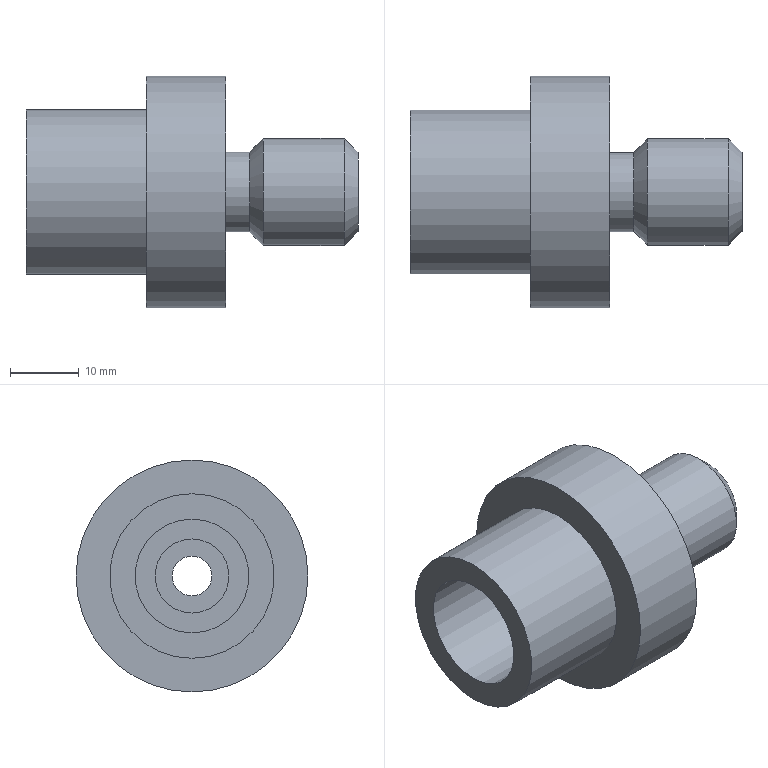Component | NX | VALVE_PORT | 1 solid | 15 faces | box 48.4 x 33.8 x 33.8 mm | volume 16682 mm3 | cylinder 7 | plane 6 | cone 2 | commonest cylinder face diameters 5.8 x1 10.8 x1 16.6 x1 24 x1 33.8 x1 11.6 x1 15.6 x1
STEP:
#1=CARTESIAN_POINT('',(0.,0.,0.));
#2=DIRECTION('',(0.,0.,1.));
#3=DIRECTION('',(1.,0.,0.));
#4=AXIS2_PLACEMENT_3D('',#1,#2,#3);
#5=CARTESIAN_POINT('',(119.195,-20.891,-5.8));
#6=VERTEX_POINT('',#5);
#7=CARTESIAN_POINT('',(119.195,-20.891,0.));
#8=DIRECTION('',(1.,0.,0.));
#9=DIRECTION('',(0.,0.,-1.));
#10=AXIS2_PLACEMENT_3D('',#7,#8,#9);
#11=CIRCLE('',#10,5.8);
#12=CARTESIAN_POINT('',(119.195,-28.691,0.));
#13=DIRECTION('',(-1.,0.,0.));
#14=DIRECTION('',(0.,0.,-1.));
#15=AXIS2_PLACEMENT_3D('',#12,#13,#14);
#16=PLANE('',#15);
#17=CARTESIAN_POINT('',(5.8,-7.8));
#18=CARTESIAN_POINT('',(5.8,-17.846));
#19=CARTESIAN_POINT('',(-2.9,-12.823));
#20=CARTESIAN_POINT('',(-11.6,-7.8));
#21=CARTESIAN_POINT('',(-2.9,-2.777));
#22=CARTESIAN_POINT('',(5.8,2.246));
#23=CARTESIAN_POINT('',(5.8,-7.8));
#24=(BOUNDED_CURVE()B_SPLINE_CURVE(2,(#17,#18,#19,#20,#21,#22,#23),.UNSPECIFIED.,.T.,.F.)B_SPLINE_CURVE_WITH_KNOTS((1,2,2,2,2,1),(-2.094,0.,2.094,4.189,6.283,8.378),.UNSPECIFIED.)CURVE()GEOMETRIC_REPRESENTATION_ITEM()RATIONAL_B_SPLINE_CURVE((1.,0.5,1.,0.5,1.,0.5,1.))REPRESENTATION_ITEM(''));
#25=(GEOMETRIC_REPRESENTATION_CONTEXT(2)PARAMETRIC_REPRESENTATION_CONTEXT()REPRESENTATION_CONTEXT('',''));
#26=DEFINITIONAL_REPRESENTATION('',(#24),#25);
#27=PCURVE('',#16,#26);
#28=CARTESIAN_POINT('',(119.195,-20.891,0.));
#29=DIRECTION('',(-1.,0.,0.));
#30=DIRECTION('',(0.,0.,-1.));
#31=AXIS2_PLACEMENT_3D('',#28,#29,#30);
#32=CONICAL_SURFACE('',#31,5.8,0.7854);
#33=CARTESIAN_POINT('',(6.283,0.));
#34=DIRECTION('',(-1.,0.));
#35=VECTOR('',#34,1.);
#36=LINE('',#33,#35);
#37=(GEOMETRIC_REPRESENTATION_CONTEXT(2)PARAMETRIC_REPRESENTATION_CONTEXT()REPRESENTATION_CONTEXT('',''));
#38=DEFINITIONAL_REPRESENTATION('',(#36),#37);
#39=PCURVE('',#32,#38);
#40=SURFACE_CURVE('',#11,(#27,#39),.PCURVE_S1.);
#41=EDGE_CURVE('',#6,#6,#40,.T.);
#42=ORIENTED_EDGE('',*,*,#41,.T.);
#43=EDGE_LOOP('',(#42));
#44=FACE_BOUND('',#43,.T.);
#45=CARTESIAN_POINT('',(119.195,-20.891,2.9));
#46=VERTEX_POINT('',#45);
#47=CARTESIAN_POINT('',(119.195,-20.891,0.));
#48=DIRECTION('',(1.,0.,0.));
#49=DIRECTION('',(0.,0.,1.));
#50=AXIS2_PLACEMENT_3D('',#47,#48,#49);
#51=CIRCLE('',#50,2.9);
#52=CARTESIAN_POINT('',(-2.9,-7.8));
#53=CARTESIAN_POINT('',(-2.9,-2.777));
#54=CARTESIAN_POINT('',(1.45,-5.289));
#55=CARTESIAN_POINT('',(5.8,-7.8));
#56=CARTESIAN_POINT('',(1.45,-10.311));
#57=CARTESIAN_POINT('',(-2.9,-12.823));
#58=CARTESIAN_POINT('',(-2.9,-7.8));
#59=(BOUNDED_CURVE()B_SPLINE_CURVE(2,(#52,#53,#54,#55,#56,#57,#58),.UNSPECIFIED.,.T.,.F.)B_SPLINE_CURVE_WITH_KNOTS((1,2,2,2,2,1),(-2.094,0.,2.094,4.189,6.283,8.378),.UNSPECIFIED.)CURVE()GEOMETRIC_REPRESENTATION_ITEM()RATIONAL_B_SPLINE_CURVE((1.,0.5,1.,0.5,1.,0.5,1.))REPRESENTATION_ITEM(''));
#60=(GEOMETRIC_REPRESENTATION_CONTEXT(2)PARAMETRIC_REPRESENTATION_CONTEXT()REPRESENTATION_CONTEXT('',''));
#61=DEFINITIONAL_REPRESENTATION('',(#59),#60);
#62=PCURVE('',#16,#61);
#63=CARTESIAN_POINT('',(70.795,-20.891,0.));
#64=DIRECTION('',(1.,0.,0.));
#65=DIRECTION('',(0.,0.,1.));
#66=AXIS2_PLACEMENT_3D('',#63,#64,#65);
#67=CYLINDRICAL_SURFACE('',#66,2.9);
#68=CARTESIAN_POINT('',(0.,48.4));
#69=DIRECTION('',(1.,0.));
#70=VECTOR('',#69,1.);
#71=LINE('',#68,#70);
#72=(GEOMETRIC_REPRESENTATION_CONTEXT(2)PARAMETRIC_REPRESENTATION_CONTEXT()REPRESENTATION_CONTEXT('',''));
#73=DEFINITIONAL_REPRESENTATION('',(#71),#72);
#74=PCURVE('',#67,#73);
#75=SURFACE_CURVE('',#51,(#62,#74),.PCURVE_S1.);
#76=EDGE_CURVE('',#46,#46,#75,.T.);
#77=ORIENTED_EDGE('',*,*,#76,.F.);
#78=EDGE_LOOP('',(#77));
#79=FACE_BOUND('',#78,.T.);
#80=ADVANCED_FACE('',(#44,#79),#16,.F.);
#81=CARTESIAN_POINT('',(88.295,-20.891,2.9));
#82=VERTEX_POINT('',#81);
#83=CARTESIAN_POINT('',(88.295,-20.891,0.));
#84=DIRECTION('',(1.,0.,0.));
#85=DIRECTION('',(0.,0.,1.));
#86=AXIS2_PLACEMENT_3D('',#83,#84,#85);
#87=CIRCLE('',#86,2.9);
#88=CARTESIAN_POINT('',(0.,17.5));
#89=DIRECTION('',(1.,0.));
#90=VECTOR('',#89,1.);
#91=LINE('',#88,#90);
#92=(GEOMETRIC_REPRESENTATION_CONTEXT(2)PARAMETRIC_REPRESENTATION_CONTEXT()REPRESENTATION_CONTEXT('',''));
#93=DEFINITIONAL_REPRESENTATION('',(#91),#92);
#94=PCURVE('',#67,#93);
#95=CARTESIAN_POINT('',(88.295,-23.791,0.));
#96=DIRECTION('',(1.,0.,0.));
#97=DIRECTION('',(0.,0.,1.));
#98=AXIS2_PLACEMENT_3D('',#95,#96,#97);
#99=PLANE('',#98);
#100=CARTESIAN_POINT('',(0.,-2.9));
#101=DIRECTION('',(1.,0.));
#102=AXIS2_PLACEMENT_2D('',#100,#101);
#103=CIRCLE('',#102,2.9);
#104=(GEOMETRIC_REPRESENTATION_CONTEXT(2)PARAMETRIC_REPRESENTATION_CONTEXT()REPRESENTATION_CONTEXT('',''));
#105=DEFINITIONAL_REPRESENTATION('',(#103),#104);
#106=PCURVE('',#99,#105);
#107=SURFACE_CURVE('',#87,(#94,#106),.PCURVE_S1.);
#108=EDGE_CURVE('',#82,#82,#107,.T.);
#109=ORIENTED_EDGE('',*,*,#108,.T.);
#110=CARTESIAN_POINT('',(88.295,-20.891,2.9));
#111=CARTESIAN_POINT('',(119.195,-20.891,2.9));
#112=B_SPLINE_CURVE_WITH_KNOTS('',1,(#110,#111),.UNSPECIFIED.,.F.,.F.,(2,2),(17.5,48.4),.PIECEWISE_BEZIER_KNOTS.);
#113=CARTESIAN_POINT('',(6.283,0.));
#114=DIRECTION('',(0.,1.));
#115=VECTOR('',#114,1.);
#116=LINE('',#113,#115);
#117=(GEOMETRIC_REPRESENTATION_CONTEXT(2)PARAMETRIC_REPRESENTATION_CONTEXT()REPRESENTATION_CONTEXT('',''));
#118=DEFINITIONAL_REPRESENTATION('',(#116),#117);
#119=PCURVE('',#67,#118);
#120=CARTESIAN_POINT('',(0.,0.));
#121=DIRECTION('',(0.,1.));
#122=VECTOR('',#121,1.);
#123=LINE('',#120,#122);
#124=(GEOMETRIC_REPRESENTATION_CONTEXT(2)PARAMETRIC_REPRESENTATION_CONTEXT()REPRESENTATION_CONTEXT('',''));
#125=DEFINITIONAL_REPRESENTATION('',(#123),#124);
#126=PCURVE('',#67,#125);
#127=SEAM_CURVE('',#112,(#119,#126),.PCURVE_S1.);
#128=EDGE_CURVE('',#82,#46,#127,.T.);
#129=ORIENTED_EDGE('',*,*,#128,.T.);
#130=ORIENTED_EDGE('',*,*,#76,.F.);
#131=ORIENTED_EDGE('',*,*,#128,.F.);
#132=EDGE_LOOP('',(#109,#129,#130,#131));
#133=FACE_BOUND('',#132,.F.);
#134=ADVANCED_FACE('',(#133),#67,.F.);
#135=CARTESIAN_POINT('',(88.295,-20.891,5.4));
#136=VERTEX_POINT('',#135);
#137=CARTESIAN_POINT('',(88.295,-20.891,0.));
#138=DIRECTION('',(1.,0.,0.));
#139=DIRECTION('',(0.,0.,1.));
#140=AXIS2_PLACEMENT_3D('',#137,#138,#139);
#141=CIRCLE('',#140,5.4);
#142=CARTESIAN_POINT('',(0.,-2.9));
#143=DIRECTION('',(1.,0.));
#144=AXIS2_PLACEMENT_2D('',#142,#143);
#145=CIRCLE('',#144,5.4);
#146=(GEOMETRIC_REPRESENTATION_CONTEXT(2)PARAMETRIC_REPRESENTATION_CONTEXT()REPRESENTATION_CONTEXT('',''));
#147=DEFINITIONAL_REPRESENTATION('',(#145),#146);
#148=PCURVE('',#99,#147);
#149=CARTESIAN_POINT('',(70.795,-20.891,0.));
#150=DIRECTION('',(1.,0.,0.));
#151=DIRECTION('',(0.,0.,1.));
#152=AXIS2_PLACEMENT_3D('',#149,#150,#151);
#153=CYLINDRICAL_SURFACE('',#152,5.4);
#154=CARTESIAN_POINT('',(0.,17.5));
#155=DIRECTION('',(1.,0.));
#156=VECTOR('',#155,1.);
#157=LINE('',#154,#156);
#158=(GEOMETRIC_REPRESENTATION_CONTEXT(2)PARAMETRIC_REPRESENTATION_CONTEXT()REPRESENTATION_CONTEXT('',''));
#159=DEFINITIONAL_REPRESENTATION('',(#157),#158);
#160=PCURVE('',#153,#159);
#161=SURFACE_CURVE('',#141,(#148,#160),.PCURVE_S1.);
#162=EDGE_CURVE('',#136,#136,#161,.T.);
#163=ORIENTED_EDGE('',*,*,#162,.F.);
#164=EDGE_LOOP('',(#163));
#165=FACE_BOUND('',#164,.T.);
#166=ORIENTED_EDGE('',*,*,#108,.T.);
#167=EDGE_LOOP('',(#166));
#168=FACE_BOUND('',#167,.T.);
#169=ADVANCED_FACE('',(#165,#168),#99,.F.);
#170=CARTESIAN_POINT('',(90.295,-20.891,5.4));
#171=VERTEX_POINT('',#170);
#172=CARTESIAN_POINT('',(90.295,-20.891,0.));
#173=DIRECTION('',(1.,0.,0.));
#174=DIRECTION('',(0.,0.,1.));
#175=AXIS2_PLACEMENT_3D('',#172,#173,#174);
#176=CIRCLE('',#175,5.4);
#177=CARTESIAN_POINT('',(0.,19.5));
#178=DIRECTION('',(1.,0.));
#179=VECTOR('',#178,1.);
#180=LINE('',#177,#179);
#181=(GEOMETRIC_REPRESENTATION_CONTEXT(2)PARAMETRIC_REPRESENTATION_CONTEXT()REPRESENTATION_CONTEXT('',''));
#182=DEFINITIONAL_REPRESENTATION('',(#180),#181);
#183=PCURVE('',#153,#182);
#184=CARTESIAN_POINT('',(90.295,-26.291,0.));
#185=DIRECTION('',(1.,0.,0.));
#186=DIRECTION('',(0.,0.,1.));
#187=AXIS2_PLACEMENT_3D('',#184,#185,#186);
#188=PLANE('',#187);
#189=CARTESIAN_POINT('',(0.,-5.4));
#190=DIRECTION('',(1.,0.));
#191=AXIS2_PLACEMENT_2D('',#189,#190);
#192=CIRCLE('',#191,5.4);
#193=(GEOMETRIC_REPRESENTATION_CONTEXT(2)PARAMETRIC_REPRESENTATION_CONTEXT()REPRESENTATION_CONTEXT('',''));
#194=DEFINITIONAL_REPRESENTATION('',(#192),#193);
#195=PCURVE('',#188,#194);
#196=SURFACE_CURVE('',#176,(#183,#195),.PCURVE_S1.);
#197=EDGE_CURVE('',#171,#171,#196,.T.);
#198=ORIENTED_EDGE('',*,*,#197,.F.);
#199=CARTESIAN_POINT('',(88.295,-20.891,5.4));
#200=CARTESIAN_POINT('',(90.295,-20.891,5.4));
#201=B_SPLINE_CURVE_WITH_KNOTS('',1,(#199,#200),.UNSPECIFIED.,.F.,.F.,(2,2),(17.5,19.5),.PIECEWISE_BEZIER_KNOTS.);
#202=CARTESIAN_POINT('',(0.,0.));
#203=DIRECTION('',(0.,1.));
#204=VECTOR('',#203,1.);
#205=LINE('',#202,#204);
#206=(GEOMETRIC_REPRESENTATION_CONTEXT(2)PARAMETRIC_REPRESENTATION_CONTEXT()REPRESENTATION_CONTEXT('',''));
#207=DEFINITIONAL_REPRESENTATION('',(#205),#206);
#208=PCURVE('',#153,#207);
#209=CARTESIAN_POINT('',(6.283,0.));
#210=DIRECTION('',(0.,1.));
#211=VECTOR('',#210,1.);
#212=LINE('',#209,#211);
#213=(GEOMETRIC_REPRESENTATION_CONTEXT(2)PARAMETRIC_REPRESENTATION_CONTEXT()REPRESENTATION_CONTEXT('',''));
#214=DEFINITIONAL_REPRESENTATION('',(#212),#213);
#215=PCURVE('',#153,#214);
#216=SEAM_CURVE('',#201,(#208,#215),.PCURVE_S1.);
#217=EDGE_CURVE('',#136,#171,#216,.T.);
#218=ORIENTED_EDGE('',*,*,#217,.F.);
#219=ORIENTED_EDGE('',*,*,#162,.T.);
#220=ORIENTED_EDGE('',*,*,#217,.T.);
#221=EDGE_LOOP('',(#198,#218,#219,#220));
#222=FACE_BOUND('',#221,.T.);
#223=ADVANCED_FACE('',(#222),#153,.T.);
#224=CARTESIAN_POINT('',(90.295,-20.891,8.3));
#225=VERTEX_POINT('',#224);
#226=CARTESIAN_POINT('',(90.295,-20.891,0.));
#227=DIRECTION('',(1.,0.,0.));
#228=DIRECTION('',(0.,0.,1.));
#229=AXIS2_PLACEMENT_3D('',#226,#227,#228);
#230=CIRCLE('',#229,8.3);
#231=CARTESIAN_POINT('',(0.,-5.4));
#232=DIRECTION('',(1.,0.));
#233=AXIS2_PLACEMENT_2D('',#231,#232);
#234=CIRCLE('',#233,8.3);
#235=(GEOMETRIC_REPRESENTATION_CONTEXT(2)PARAMETRIC_REPRESENTATION_CONTEXT()REPRESENTATION_CONTEXT('',''));
#236=DEFINITIONAL_REPRESENTATION('',(#234),#235);
#237=PCURVE('',#188,#236);
#238=CARTESIAN_POINT('',(70.795,-20.891,0.));
#239=DIRECTION('',(1.,0.,0.));
#240=DIRECTION('',(0.,0.,1.));
#241=AXIS2_PLACEMENT_3D('',#238,#239,#240);
#242=CYLINDRICAL_SURFACE('',#241,8.3);
#243=CARTESIAN_POINT('',(0.,19.5));
#244=DIRECTION('',(1.,0.));
#245=VECTOR('',#244,1.);
#246=LINE('',#243,#245);
#247=(GEOMETRIC_REPRESENTATION_CONTEXT(2)PARAMETRIC_REPRESENTATION_CONTEXT()REPRESENTATION_CONTEXT('',''));
#248=DEFINITIONAL_REPRESENTATION('',(#246),#247);
#249=PCURVE('',#242,#248);
#250=SURFACE_CURVE('',#230,(#237,#249),.PCURVE_S1.);
#251=EDGE_CURVE('',#225,#225,#250,.T.);
#252=ORIENTED_EDGE('',*,*,#251,.F.);
#253=EDGE_LOOP('',(#252));
#254=FACE_BOUND('',#253,.T.);
#255=ORIENTED_EDGE('',*,*,#197,.T.);
#256=EDGE_LOOP('',(#255));
#257=FACE_BOUND('',#256,.T.);
#258=ADVANCED_FACE('',(#254,#257),#188,.F.);
#259=CARTESIAN_POINT('',(70.795,-20.891,8.3));
#260=VERTEX_POINT('',#259);
#261=CARTESIAN_POINT('',(70.795,-20.891,0.));
#262=DIRECTION('',(1.,0.,0.));
#263=DIRECTION('',(0.,0.,1.));
#264=AXIS2_PLACEMENT_3D('',#261,#262,#263);
#265=CIRCLE('',#264,8.3);
#266=CARTESIAN_POINT('',(0.,0.));
#267=DIRECTION('',(1.,0.));
#268=VECTOR('',#267,1.);
#269=LINE('',#266,#268);
#270=(GEOMETRIC_REPRESENTATION_CONTEXT(2)PARAMETRIC_REPRESENTATION_CONTEXT()REPRESENTATION_CONTEXT('',''));
#271=DEFINITIONAL_REPRESENTATION('',(#269),#270);
#272=PCURVE('',#242,#271);
#273=CARTESIAN_POINT('',(70.795,-29.191,0.));
#274=DIRECTION('',(1.,0.,0.));
#275=DIRECTION('',(0.,0.,1.));
#276=AXIS2_PLACEMENT_3D('',#273,#274,#275);
#277=PLANE('',#276);
#278=CARTESIAN_POINT('',(0.,-8.3));
#279=DIRECTION('',(1.,0.));
#280=AXIS2_PLACEMENT_2D('',#278,#279);
#281=CIRCLE('',#280,8.3);
#282=(GEOMETRIC_REPRESENTATION_CONTEXT(2)PARAMETRIC_REPRESENTATION_CONTEXT()REPRESENTATION_CONTEXT('',''));
#283=DEFINITIONAL_REPRESENTATION('',(#281),#282);
#284=PCURVE('',#277,#283);
#285=SURFACE_CURVE('',#265,(#272,#284),.PCURVE_S1.);
#286=EDGE_CURVE('',#260,#260,#285,.T.);
#287=ORIENTED_EDGE('',*,*,#286,.T.);
#288=CARTESIAN_POINT('',(70.795,-20.891,8.3));
#289=CARTESIAN_POINT('',(90.295,-20.891,8.3));
#290=B_SPLINE_CURVE_WITH_KNOTS('',1,(#288,#289),.UNSPECIFIED.,.F.,.F.,(2,2),(0.,19.5),.PIECEWISE_BEZIER_KNOTS.);
#291=CARTESIAN_POINT('',(6.283,0.));
#292=DIRECTION('',(0.,1.));
#293=VECTOR('',#292,1.);
#294=LINE('',#291,#293);
#295=(GEOMETRIC_REPRESENTATION_CONTEXT(2)PARAMETRIC_REPRESENTATION_CONTEXT()REPRESENTATION_CONTEXT('',''));
#296=DEFINITIONAL_REPRESENTATION('',(#294),#295);
#297=PCURVE('',#242,#296);
#298=CARTESIAN_POINT('',(0.,0.));
#299=DIRECTION('',(0.,1.));
#300=VECTOR('',#299,1.);
#301=LINE('',#298,#300);
#302=(GEOMETRIC_REPRESENTATION_CONTEXT(2)PARAMETRIC_REPRESENTATION_CONTEXT()REPRESENTATION_CONTEXT('',''));
#303=DEFINITIONAL_REPRESENTATION('',(#301),#302);
#304=PCURVE('',#242,#303);
#305=SEAM_CURVE('',#290,(#297,#304),.PCURVE_S1.);
#306=EDGE_CURVE('',#260,#225,#305,.T.);
#307=ORIENTED_EDGE('',*,*,#306,.T.);
#308=ORIENTED_EDGE('',*,*,#251,.F.);
#309=ORIENTED_EDGE('',*,*,#306,.F.);
#310=EDGE_LOOP('',(#287,#307,#308,#309));
#311=FACE_BOUND('',#310,.F.);
#312=ADVANCED_FACE('',(#311),#242,.F.);
#313=CARTESIAN_POINT('',(70.795,-20.891,12.));
#314=VERTEX_POINT('',#313);
#315=CARTESIAN_POINT('',(70.795,-20.891,0.));
#316=DIRECTION('',(1.,0.,0.));
#317=DIRECTION('',(0.,0.,1.));
#318=AXIS2_PLACEMENT_3D('',#315,#316,#317);
#319=CIRCLE('',#318,12.);
#320=CARTESIAN_POINT('',(0.,-8.3));
#321=DIRECTION('',(1.,0.));
#322=AXIS2_PLACEMENT_2D('',#320,#321);
#323=CIRCLE('',#322,12.);
#324=(GEOMETRIC_REPRESENTATION_CONTEXT(2)PARAMETRIC_REPRESENTATION_CONTEXT()REPRESENTATION_CONTEXT('',''));
#325=DEFINITIONAL_REPRESENTATION('',(#323),#324);
#326=PCURVE('',#277,#325);
#327=CARTESIAN_POINT('',(70.795,-20.891,0.));
#328=DIRECTION('',(1.,0.,0.));
#329=DIRECTION('',(0.,0.,1.));
#330=AXIS2_PLACEMENT_3D('',#327,#328,#329);
#331=CYLINDRICAL_SURFACE('',#330,12.);
#332=CARTESIAN_POINT('',(0.,0.));
#333=DIRECTION('',(1.,0.));
#334=VECTOR('',#333,1.);
#335=LINE('',#332,#334);
#336=(GEOMETRIC_REPRESENTATION_CONTEXT(2)PARAMETRIC_REPRESENTATION_CONTEXT()REPRESENTATION_CONTEXT('',''));
#337=DEFINITIONAL_REPRESENTATION('',(#335),#336);
#338=PCURVE('',#331,#337);
#339=SURFACE_CURVE('',#319,(#326,#338),.PCURVE_S1.);
#340=EDGE_CURVE('',#314,#314,#339,.T.);
#341=ORIENTED_EDGE('',*,*,#340,.F.);
#342=EDGE_LOOP('',(#341));
#343=FACE_BOUND('',#342,.T.);
#344=ORIENTED_EDGE('',*,*,#286,.T.);
#345=EDGE_LOOP('',(#344));
#346=FACE_BOUND('',#345,.T.);
#347=ADVANCED_FACE('',(#343,#346),#277,.F.);
#348=CARTESIAN_POINT('',(88.295,-20.891,12.));
#349=VERTEX_POINT('',#348);
#350=CARTESIAN_POINT('',(88.295,-20.891,0.));
#351=DIRECTION('',(1.,0.,0.));
#352=DIRECTION('',(0.,0.,1.));
#353=AXIS2_PLACEMENT_3D('',#350,#351,#352);
#354=CIRCLE('',#353,12.);
#355=CARTESIAN_POINT('',(0.,17.5));
#356=DIRECTION('',(1.,0.));
#357=VECTOR('',#356,1.);
#358=LINE('',#355,#357);
#359=(GEOMETRIC_REPRESENTATION_CONTEXT(2)PARAMETRIC_REPRESENTATION_CONTEXT()REPRESENTATION_CONTEXT('',''));
#360=DEFINITIONAL_REPRESENTATION('',(#358),#359);
#361=PCURVE('',#331,#360);
#362=CARTESIAN_POINT('',(88.295,-32.891,0.));
#363=DIRECTION('',(1.,0.,0.));
#364=DIRECTION('',(0.,0.,1.));
#365=AXIS2_PLACEMENT_3D('',#362,#363,#364);
#366=PLANE('',#365);
#367=CARTESIAN_POINT('',(0.,-12.));
#368=DIRECTION('',(1.,0.));
#369=AXIS2_PLACEMENT_2D('',#367,#368);
#370=CIRCLE('',#369,12.);
#371=(GEOMETRIC_REPRESENTATION_CONTEXT(2)PARAMETRIC_REPRESENTATION_CONTEXT()REPRESENTATION_CONTEXT('',''));
#372=DEFINITIONAL_REPRESENTATION('',(#370),#371);
#373=PCURVE('',#366,#372);
#374=SURFACE_CURVE('',#354,(#361,#373),.PCURVE_S1.);
#375=EDGE_CURVE('',#349,#349,#374,.T.);
#376=ORIENTED_EDGE('',*,*,#375,.F.);
#377=CARTESIAN_POINT('',(70.795,-20.891,12.));
#378=CARTESIAN_POINT('',(88.295,-20.891,12.));
#379=B_SPLINE_CURVE_WITH_KNOTS('',1,(#377,#378),.UNSPECIFIED.,.F.,.F.,(2,2),(0.,17.5),.PIECEWISE_BEZIER_KNOTS.);
#380=CARTESIAN_POINT('',(0.,0.));
#381=DIRECTION('',(0.,1.));
#382=VECTOR('',#381,1.);
#383=LINE('',#380,#382);
#384=(GEOMETRIC_REPRESENTATION_CONTEXT(2)PARAMETRIC_REPRESENTATION_CONTEXT()REPRESENTATION_CONTEXT('',''));
#385=DEFINITIONAL_REPRESENTATION('',(#383),#384);
#386=PCURVE('',#331,#385);
#387=CARTESIAN_POINT('',(6.283,0.));
#388=DIRECTION('',(0.,1.));
#389=VECTOR('',#388,1.);
#390=LINE('',#387,#389);
#391=(GEOMETRIC_REPRESENTATION_CONTEXT(2)PARAMETRIC_REPRESENTATION_CONTEXT()REPRESENTATION_CONTEXT('',''));
#392=DEFINITIONAL_REPRESENTATION('',(#390),#391);
#393=PCURVE('',#331,#392);
#394=SEAM_CURVE('',#379,(#386,#393),.PCURVE_S1.);
#395=EDGE_CURVE('',#314,#349,#394,.T.);
#396=ORIENTED_EDGE('',*,*,#395,.F.);
#397=ORIENTED_EDGE('',*,*,#340,.T.);
#398=ORIENTED_EDGE('',*,*,#395,.T.);
#399=EDGE_LOOP('',(#376,#396,#397,#398));
#400=FACE_BOUND('',#399,.T.);
#401=ADVANCED_FACE('',(#400),#331,.T.);
#402=CARTESIAN_POINT('',(88.295,-20.891,16.9));
#403=VERTEX_POINT('',#402);
#404=CARTESIAN_POINT('',(88.295,-20.891,0.));
#405=DIRECTION('',(1.,0.,0.));
#406=DIRECTION('',(0.,0.,1.));
#407=AXIS2_PLACEMENT_3D('',#404,#405,#406);
#408=CIRCLE('',#407,16.9);
#409=CARTESIAN_POINT('',(0.,-12.));
#410=DIRECTION('',(1.,0.));
#411=AXIS2_PLACEMENT_2D('',#409,#410);
#412=CIRCLE('',#411,16.9);
#413=(GEOMETRIC_REPRESENTATION_CONTEXT(2)PARAMETRIC_REPRESENTATION_CONTEXT()REPRESENTATION_CONTEXT('',''));
#414=DEFINITIONAL_REPRESENTATION('',(#412),#413);
#415=PCURVE('',#366,#414);
#416=CARTESIAN_POINT('',(70.795,-20.891,0.));
#417=DIRECTION('',(1.,0.,0.));
#418=DIRECTION('',(0.,0.,1.));
#419=AXIS2_PLACEMENT_3D('',#416,#417,#418);
#420=CYLINDRICAL_SURFACE('',#419,16.9);
#421=CARTESIAN_POINT('',(0.,17.5));
#422=DIRECTION('',(1.,0.));
#423=VECTOR('',#422,1.);
#424=LINE('',#421,#423);
#425=(GEOMETRIC_REPRESENTATION_CONTEXT(2)PARAMETRIC_REPRESENTATION_CONTEXT()REPRESENTATION_CONTEXT('',''));
#426=DEFINITIONAL_REPRESENTATION('',(#424),#425);
#427=PCURVE('',#420,#426);
#428=SURFACE_CURVE('',#408,(#415,#427),.PCURVE_S1.);
#429=EDGE_CURVE('',#403,#403,#428,.T.);
#430=ORIENTED_EDGE('',*,*,#429,.F.);
#431=EDGE_LOOP('',(#430));
#432=FACE_BOUND('',#431,.T.);
#433=ORIENTED_EDGE('',*,*,#375,.T.);
#434=EDGE_LOOP('',(#433));
#435=FACE_BOUND('',#434,.T.);
#436=ADVANCED_FACE('',(#432,#435),#366,.F.);
#437=CARTESIAN_POINT('',(99.895,-20.891,16.9));
#438=VERTEX_POINT('',#437);
#439=CARTESIAN_POINT('',(99.895,-20.891,0.));
#440=DIRECTION('',(1.,0.,0.));
#441=DIRECTION('',(0.,0.,1.));
#442=AXIS2_PLACEMENT_3D('',#439,#440,#441);
#443=CIRCLE('',#442,16.9);
#444=CARTESIAN_POINT('',(0.,29.1));
#445=DIRECTION('',(1.,0.));
#446=VECTOR('',#445,1.);
#447=LINE('',#444,#446);
#448=(GEOMETRIC_REPRESENTATION_CONTEXT(2)PARAMETRIC_REPRESENTATION_CONTEXT()REPRESENTATION_CONTEXT('',''));
#449=DEFINITIONAL_REPRESENTATION('',(#447),#448);
#450=PCURVE('',#420,#449);
#451=CARTESIAN_POINT('',(99.895,-37.791,0.));
#452=DIRECTION('',(-1.,0.,0.));
#453=DIRECTION('',(0.,0.,-1.));
#454=AXIS2_PLACEMENT_3D('',#451,#452,#453);
#455=PLANE('',#454);
#456=CARTESIAN_POINT('',(-16.9,-16.9));
#457=CARTESIAN_POINT('',(-16.9,12.372));
#458=CARTESIAN_POINT('',(8.45,-2.264));
#459=CARTESIAN_POINT('',(33.8,-16.9));
#460=CARTESIAN_POINT('',(8.45,-31.536));
#461=CARTESIAN_POINT('',(-16.9,-46.172));
#462=CARTESIAN_POINT('',(-16.9,-16.9));
#463=(BOUNDED_CURVE()B_SPLINE_CURVE(2,(#456,#457,#458,#459,#460,#461,#462),.UNSPECIFIED.,.T.,.F.)B_SPLINE_CURVE_WITH_KNOTS((1,2,2,2,2,1),(-2.094,0.,2.094,4.189,6.283,8.378),.UNSPECIFIED.)CURVE()GEOMETRIC_REPRESENTATION_ITEM()RATIONAL_B_SPLINE_CURVE((1.,0.5,1.,0.5,1.,0.5,1.))REPRESENTATION_ITEM(''));
#464=(GEOMETRIC_REPRESENTATION_CONTEXT(2)PARAMETRIC_REPRESENTATION_CONTEXT()REPRESENTATION_CONTEXT('',''));
#465=DEFINITIONAL_REPRESENTATION('',(#463),#464);
#466=PCURVE('',#455,#465);
#467=SURFACE_CURVE('',#443,(#450,#466),.PCURVE_S1.);
#468=EDGE_CURVE('',#438,#438,#467,.T.);
#469=ORIENTED_EDGE('',*,*,#468,.F.);
#470=CARTESIAN_POINT('',(88.295,-20.891,16.9));
#471=CARTESIAN_POINT('',(99.895,-20.891,16.9));
#472=B_SPLINE_CURVE_WITH_KNOTS('',1,(#470,#471),.UNSPECIFIED.,.F.,.F.,(2,2),(17.5,29.1),.PIECEWISE_BEZIER_KNOTS.);
#473=CARTESIAN_POINT('',(0.,0.));
#474=DIRECTION('',(0.,1.));
#475=VECTOR('',#474,1.);
#476=LINE('',#473,#475);
#477=(GEOMETRIC_REPRESENTATION_CONTEXT(2)PARAMETRIC_REPRESENTATION_CONTEXT()REPRESENTATION_CONTEXT('',''));
#478=DEFINITIONAL_REPRESENTATION('',(#476),#477);
#479=PCURVE('',#420,#478);
#480=CARTESIAN_POINT('',(6.283,0.));
#481=DIRECTION('',(0.,1.));
#482=VECTOR('',#481,1.);
#483=LINE('',#480,#482);
#484=(GEOMETRIC_REPRESENTATION_CONTEXT(2)PARAMETRIC_REPRESENTATION_CONTEXT()REPRESENTATION_CONTEXT('',''));
#485=DEFINITIONAL_REPRESENTATION('',(#483),#484);
#486=PCURVE('',#420,#485);
#487=SEAM_CURVE('',#472,(#479,#486),.PCURVE_S1.);
#488=EDGE_CURVE('',#403,#438,#487,.T.);
#489=ORIENTED_EDGE('',*,*,#488,.F.);
#490=ORIENTED_EDGE('',*,*,#429,.T.);
#491=ORIENTED_EDGE('',*,*,#488,.T.);
#492=EDGE_LOOP('',(#469,#489,#490,#491));
#493=FACE_BOUND('',#492,.T.);
#494=ADVANCED_FACE('',(#493),#420,.T.);
#495=CARTESIAN_POINT('',(99.895,-20.891,5.8));
#496=VERTEX_POINT('',#495);
#497=CARTESIAN_POINT('',(99.895,-20.891,0.));
#498=DIRECTION('',(1.,0.,0.));
#499=DIRECTION('',(0.,0.,1.));
#500=AXIS2_PLACEMENT_3D('',#497,#498,#499);
#501=CIRCLE('',#500,5.8);
#502=CARTESIAN_POINT('',(-5.8,-16.9));
#503=CARTESIAN_POINT('',(-5.8,-6.854));
#504=CARTESIAN_POINT('',(2.9,-11.877));
#505=CARTESIAN_POINT('',(11.6,-16.9));
#506=CARTESIAN_POINT('',(2.9,-21.923));
#507=CARTESIAN_POINT('',(-5.8,-26.946));
#508=CARTESIAN_POINT('',(-5.8,-16.9));
#509=(BOUNDED_CURVE()B_SPLINE_CURVE(2,(#502,#503,#504,#505,#506,#507,#508),.UNSPECIFIED.,.T.,.F.)B_SPLINE_CURVE_WITH_KNOTS((1,2,2,2,2,1),(-2.094,0.,2.094,4.189,6.283,8.378),.UNSPECIFIED.)CURVE()GEOMETRIC_REPRESENTATION_ITEM()RATIONAL_B_SPLINE_CURVE((1.,0.5,1.,0.5,1.,0.5,1.))REPRESENTATION_ITEM(''));
#510=(GEOMETRIC_REPRESENTATION_CONTEXT(2)PARAMETRIC_REPRESENTATION_CONTEXT()REPRESENTATION_CONTEXT('',''));
#511=DEFINITIONAL_REPRESENTATION('',(#509),#510);
#512=PCURVE('',#455,#511);
#513=CARTESIAN_POINT('',(70.795,-20.891,0.));
#514=DIRECTION('',(1.,0.,0.));
#515=DIRECTION('',(0.,0.,1.));
#516=AXIS2_PLACEMENT_3D('',#513,#514,#515);
#517=CYLINDRICAL_SURFACE('',#516,5.8);
#518=CARTESIAN_POINT('',(0.,29.1));
#519=DIRECTION('',(1.,0.));
#520=VECTOR('',#519,1.);
#521=LINE('',#518,#520);
#522=(GEOMETRIC_REPRESENTATION_CONTEXT(2)PARAMETRIC_REPRESENTATION_CONTEXT()REPRESENTATION_CONTEXT('',''));
#523=DEFINITIONAL_REPRESENTATION('',(#521),#522);
#524=PCURVE('',#517,#523);
#525=SURFACE_CURVE('',#501,(#512,#524),.PCURVE_S1.);
#526=EDGE_CURVE('',#496,#496,#525,.T.);
#527=ORIENTED_EDGE('',*,*,#526,.F.);
#528=EDGE_LOOP('',(#527));
#529=FACE_BOUND('',#528,.T.);
#530=ORIENTED_EDGE('',*,*,#468,.T.);
#531=EDGE_LOOP('',(#530));
#532=FACE_BOUND('',#531,.T.);
#533=ADVANCED_FACE('',(#529,#532),#455,.F.);
#534=CARTESIAN_POINT('',(103.395,-20.891,5.8));
#535=VERTEX_POINT('',#534);
#536=CARTESIAN_POINT('',(103.395,-20.891,0.));
#537=DIRECTION('',(1.,0.,0.));
#538=DIRECTION('',(0.,0.,1.));
#539=AXIS2_PLACEMENT_3D('',#536,#537,#538);
#540=CIRCLE('',#539,5.8);
#541=CARTESIAN_POINT('',(0.,32.6));
#542=DIRECTION('',(1.,0.));
#543=VECTOR('',#542,1.);
#544=LINE('',#541,#543);
#545=(GEOMETRIC_REPRESENTATION_CONTEXT(2)PARAMETRIC_REPRESENTATION_CONTEXT()REPRESENTATION_CONTEXT('',''));
#546=DEFINITIONAL_REPRESENTATION('',(#544),#545);
#547=PCURVE('',#517,#546);
#548=CARTESIAN_POINT('',(105.395,-20.891,0.));
#549=DIRECTION('',(1.,0.,0.));
#550=DIRECTION('',(0.,0.,1.));
#551=AXIS2_PLACEMENT_3D('',#548,#549,#550);
#552=CONICAL_SURFACE('',#551,7.8,0.7854);
#553=CARTESIAN_POINT('',(0.,-2.));
#554=DIRECTION('',(1.,0.));
#555=VECTOR('',#554,1.);
#556=LINE('',#553,#555);
#557=(GEOMETRIC_REPRESENTATION_CONTEXT(2)PARAMETRIC_REPRESENTATION_CONTEXT()REPRESENTATION_CONTEXT('',''));
#558=DEFINITIONAL_REPRESENTATION('',(#556),#557);
#559=PCURVE('',#552,#558);
#560=SURFACE_CURVE('',#540,(#547,#559),.PCURVE_S1.);
#561=EDGE_CURVE('',#535,#535,#560,.T.);
#562=ORIENTED_EDGE('',*,*,#561,.F.);
#563=CARTESIAN_POINT('',(99.895,-20.891,5.8));
#564=CARTESIAN_POINT('',(103.395,-20.891,5.8));
#565=B_SPLINE_CURVE_WITH_KNOTS('',1,(#563,#564),.UNSPECIFIED.,.F.,.F.,(2,2),(29.1,32.6),.PIECEWISE_BEZIER_KNOTS.);
#566=CARTESIAN_POINT('',(0.,0.));
#567=DIRECTION('',(0.,1.));
#568=VECTOR('',#567,1.);
#569=LINE('',#566,#568);
#570=(GEOMETRIC_REPRESENTATION_CONTEXT(2)PARAMETRIC_REPRESENTATION_CONTEXT()REPRESENTATION_CONTEXT('',''));
#571=DEFINITIONAL_REPRESENTATION('',(#569),#570);
#572=PCURVE('',#517,#571);
#573=CARTESIAN_POINT('',(6.283,0.));
#574=DIRECTION('',(0.,1.));
#575=VECTOR('',#574,1.);
#576=LINE('',#573,#575);
#577=(GEOMETRIC_REPRESENTATION_CONTEXT(2)PARAMETRIC_REPRESENTATION_CONTEXT()REPRESENTATION_CONTEXT('',''));
#578=DEFINITIONAL_REPRESENTATION('',(#576),#577);
#579=PCURVE('',#517,#578);
#580=SEAM_CURVE('',#565,(#572,#579),.PCURVE_S1.);
#581=EDGE_CURVE('',#496,#535,#580,.T.);
#582=ORIENTED_EDGE('',*,*,#581,.F.);
#583=ORIENTED_EDGE('',*,*,#526,.T.);
#584=ORIENTED_EDGE('',*,*,#581,.T.);
#585=EDGE_LOOP('',(#562,#582,#583,#584));
#586=FACE_BOUND('',#585,.T.);
#587=ADVANCED_FACE('',(#586),#517,.T.);
#588=CARTESIAN_POINT('',(105.395,-20.891,7.8));
#589=VERTEX_POINT('',#588);
#590=CARTESIAN_POINT('',(105.395,-20.891,0.));
#591=DIRECTION('',(1.,0.,0.));
#592=DIRECTION('',(0.,0.,1.));
#593=AXIS2_PLACEMENT_3D('',#590,#591,#592);
#594=CIRCLE('',#593,7.8);
#595=CARTESIAN_POINT('',(70.795,-20.891,0.));
#596=DIRECTION('',(1.,0.,0.));
#597=DIRECTION('',(0.,0.,1.));
#598=AXIS2_PLACEMENT_3D('',#595,#596,#597);
#599=CYLINDRICAL_SURFACE('',#598,7.8);
#600=CARTESIAN_POINT('',(0.,34.6));
#601=DIRECTION('',(1.,0.));
#602=VECTOR('',#601,1.);
#603=LINE('',#600,#602);
#604=(GEOMETRIC_REPRESENTATION_CONTEXT(2)PARAMETRIC_REPRESENTATION_CONTEXT()REPRESENTATION_CONTEXT('',''));
#605=DEFINITIONAL_REPRESENTATION('',(#603),#604);
#606=PCURVE('',#599,#605);
#607=CARTESIAN_POINT('',(0.,0.));
#608=DIRECTION('',(1.,0.));
#609=VECTOR('',#608,1.);
#610=LINE('',#607,#609);
#611=(GEOMETRIC_REPRESENTATION_CONTEXT(2)PARAMETRIC_REPRESENTATION_CONTEXT()REPRESENTATION_CONTEXT('',''));
#612=DEFINITIONAL_REPRESENTATION('',(#610),#611);
#613=PCURVE('',#552,#612);
#614=SURFACE_CURVE('',#594,(#606,#613),.PCURVE_S1.);
#615=EDGE_CURVE('',#589,#589,#614,.T.);
#616=ORIENTED_EDGE('',*,*,#615,.T.);
#617=CARTESIAN_POINT('',(117.195,-20.891,7.8));
#618=VERTEX_POINT('',#617);
#619=CARTESIAN_POINT('',(105.395,-20.891,7.8));
#620=CARTESIAN_POINT('',(117.195,-20.891,7.8));
#621=B_SPLINE_CURVE_WITH_KNOTS('',1,(#619,#620),.UNSPECIFIED.,.F.,.F.,(2,2),(34.6,46.4),.PIECEWISE_BEZIER_KNOTS.);
#622=CARTESIAN_POINT('',(6.283,0.));
#623=DIRECTION('',(0.,1.));
#624=VECTOR('',#623,1.);
#625=LINE('',#622,#624);
#626=(GEOMETRIC_REPRESENTATION_CONTEXT(2)PARAMETRIC_REPRESENTATION_CONTEXT()REPRESENTATION_CONTEXT('',''));
#627=DEFINITIONAL_REPRESENTATION('',(#625),#626);
#628=PCURVE('',#599,#627);
#629=CARTESIAN_POINT('',(0.,0.));
#630=DIRECTION('',(0.,1.));
#631=VECTOR('',#630,1.);
#632=LINE('',#629,#631);
#633=(GEOMETRIC_REPRESENTATION_CONTEXT(2)PARAMETRIC_REPRESENTATION_CONTEXT()REPRESENTATION_CONTEXT('',''));
#634=DEFINITIONAL_REPRESENTATION('',(#632),#633);
#635=PCURVE('',#599,#634);
#636=SEAM_CURVE('',#621,(#628,#635),.PCURVE_S1.);
#637=EDGE_CURVE('',#589,#618,#636,.T.);
#638=ORIENTED_EDGE('',*,*,#637,.T.);
#639=CARTESIAN_POINT('',(117.195,-20.891,-7.8));
#640=VERTEX_POINT('',#639);
#641=CARTESIAN_POINT('',(117.195,-20.891,0.));
#642=DIRECTION('',(-1.,0.,0.));
#643=DIRECTION('',(0.,0.,-1.));
#644=AXIS2_PLACEMENT_3D('',#641,#642,#643);
#645=CIRCLE('',#644,7.8);
#646=CARTESIAN_POINT('',(9.425,46.4));
#647=DIRECTION('',(-1.,0.));
#648=VECTOR('',#647,1.);
#649=LINE('',#646,#648);
#650=(GEOMETRIC_REPRESENTATION_CONTEXT(2)PARAMETRIC_REPRESENTATION_CONTEXT()REPRESENTATION_CONTEXT('',''));
#651=DEFINITIONAL_REPRESENTATION('',(#649),#650);
#652=PCURVE('',#599,#651);
#653=CARTESIAN_POINT('',(0.,2.));
#654=DIRECTION('',(1.,0.));
#655=VECTOR('',#654,1.);
#656=LINE('',#653,#655);
#657=(GEOMETRIC_REPRESENTATION_CONTEXT(2)PARAMETRIC_REPRESENTATION_CONTEXT()REPRESENTATION_CONTEXT('',''));
#658=DEFINITIONAL_REPRESENTATION('',(#656),#657);
#659=PCURVE('',#32,#658);
#660=SURFACE_CURVE('',#645,(#652,#659),.PCURVE_S1.);
#661=EDGE_CURVE('',#618,#640,#660,.T.);
#662=ORIENTED_EDGE('',*,*,#661,.T.);
#663=CARTESIAN_POINT('',(117.195,-20.891,0.));
#664=DIRECTION('',(-1.,0.,0.));
#665=DIRECTION('',(0.,0.,-1.));
#666=AXIS2_PLACEMENT_3D('',#663,#664,#665);
#667=CIRCLE('',#666,7.8);
#668=CARTESIAN_POINT('',(3.142,46.4));
#669=DIRECTION('',(-1.,0.));
#670=VECTOR('',#669,1.);
#671=LINE('',#668,#670);
#672=(GEOMETRIC_REPRESENTATION_CONTEXT(2)PARAMETRIC_REPRESENTATION_CONTEXT()REPRESENTATION_CONTEXT('',''));
#673=DEFINITIONAL_REPRESENTATION('',(#671),#672);
#674=PCURVE('',#599,#673);
#675=CARTESIAN_POINT('',(0.,2.));
#676=DIRECTION('',(1.,0.));
#677=VECTOR('',#676,1.);
#678=LINE('',#675,#677);
#679=(GEOMETRIC_REPRESENTATION_CONTEXT(2)PARAMETRIC_REPRESENTATION_CONTEXT()REPRESENTATION_CONTEXT('',''));
#680=DEFINITIONAL_REPRESENTATION('',(#678),#679);
#681=PCURVE('',#32,#680);
#682=SURFACE_CURVE('',#667,(#674,#681),.PCURVE_S1.);
#683=EDGE_CURVE('',#640,#618,#682,.T.);
#684=ORIENTED_EDGE('',*,*,#683,.T.);
#685=ORIENTED_EDGE('',*,*,#637,.F.);
#686=EDGE_LOOP('',(#616,#638,#662,#684,#685));
#687=FACE_BOUND('',#686,.T.);
#688=ADVANCED_FACE('',(#687),#599,.T.);
#689=ORIENTED_EDGE('',*,*,#561,.T.);
#690=CARTESIAN_POINT('',(103.395,-20.891,5.8));
#691=CARTESIAN_POINT('',(105.395,-20.891,7.8));
#692=B_SPLINE_CURVE_WITH_KNOTS('',1,(#690,#691),.UNSPECIFIED.,.F.,.F.,(2,2),(-2.828,0.),.PIECEWISE_BEZIER_KNOTS.);
#693=CARTESIAN_POINT('',(6.283,0.));
#694=DIRECTION('',(0.,1.));
#695=VECTOR('',#694,1.);
#696=LINE('',#693,#695);
#697=(GEOMETRIC_REPRESENTATION_CONTEXT(2)PARAMETRIC_REPRESENTATION_CONTEXT()REPRESENTATION_CONTEXT('',''));
#698=DEFINITIONAL_REPRESENTATION('',(#696),#697);
#699=PCURVE('',#552,#698);
#700=CARTESIAN_POINT('',(0.,0.));
#701=DIRECTION('',(0.,1.));
#702=VECTOR('',#701,1.);
#703=LINE('',#700,#702);
#704=(GEOMETRIC_REPRESENTATION_CONTEXT(2)PARAMETRIC_REPRESENTATION_CONTEXT()REPRESENTATION_CONTEXT('',''));
#705=DEFINITIONAL_REPRESENTATION('',(#703),#704);
#706=PCURVE('',#552,#705);
#707=SEAM_CURVE('',#692,(#699,#706),.PCURVE_S1.);
#708=EDGE_CURVE('',#535,#589,#707,.T.);
#709=ORIENTED_EDGE('',*,*,#708,.T.);
#710=ORIENTED_EDGE('',*,*,#615,.F.);
#711=ORIENTED_EDGE('',*,*,#708,.F.);
#712=EDGE_LOOP('',(#689,#709,#710,#711));
#713=FACE_BOUND('',#712,.T.);
#714=ADVANCED_FACE('',(#713),#552,.T.);
#715=ORIENTED_EDGE('',*,*,#683,.F.);
#716=CARTESIAN_POINT('',(119.195,-20.891,-5.8));
#717=CARTESIAN_POINT('',(117.195,-20.891,-7.8));
#718=B_SPLINE_CURVE_WITH_KNOTS('',1,(#716,#717),.UNSPECIFIED.,.F.,.F.,(2,2),(0.,2.828),.PIECEWISE_BEZIER_KNOTS.);
#719=CARTESIAN_POINT('',(0.,0.));
#720=DIRECTION('',(0.,1.));
#721=VECTOR('',#720,1.);
#722=LINE('',#719,#721);
#723=(GEOMETRIC_REPRESENTATION_CONTEXT(2)PARAMETRIC_REPRESENTATION_CONTEXT()REPRESENTATION_CONTEXT('',''));
#724=DEFINITIONAL_REPRESENTATION('',(#722),#723);
#725=PCURVE('',#32,#724);
#726=CARTESIAN_POINT('',(6.283,0.));
#727=DIRECTION('',(0.,1.));
#728=VECTOR('',#727,1.);
#729=LINE('',#726,#728);
#730=(GEOMETRIC_REPRESENTATION_CONTEXT(2)PARAMETRIC_REPRESENTATION_CONTEXT()REPRESENTATION_CONTEXT('',''));
#731=DEFINITIONAL_REPRESENTATION('',(#729),#730);
#732=PCURVE('',#32,#731);
#733=SEAM_CURVE('',#718,(#725,#732),.PCURVE_S1.);
#734=EDGE_CURVE('',#6,#640,#733,.T.);
#735=ORIENTED_EDGE('',*,*,#734,.F.);
#736=ORIENTED_EDGE('',*,*,#41,.F.);
#737=ORIENTED_EDGE('',*,*,#734,.T.);
#738=ORIENTED_EDGE('',*,*,#661,.F.);
#739=EDGE_LOOP('',(#715,#735,#736,#737,#738));
#740=FACE_BOUND('',#739,.T.);
#741=ADVANCED_FACE('',(#740),#32,.T.);
#742=CLOSED_SHELL('',(#80,#134,#169,#223,#258,#312,#347,#401,#436,#494,#533,#587,#688,#714,#741));
#743=MANIFOLD_SOLID_BREP('',#742);
#744=(LENGTH_UNIT()NAMED_UNIT(*)SI_UNIT(.MILLI.,.METRE.));
#745=UNCERTAINTY_MEASURE_WITH_UNIT(LENGTH_MEASURE(0.00001),#744,'','');
#746=(NAMED_UNIT(*)PLANE_ANGLE_UNIT()SI_UNIT($,.RADIAN.));
#747=(NAMED_UNIT(*)SI_UNIT($,.STERADIAN.)SOLID_ANGLE_UNIT());
#748=(GEOMETRIC_REPRESENTATION_CONTEXT(3)GLOBAL_UNCERTAINTY_ASSIGNED_CONTEXT((#745))GLOBAL_UNIT_ASSIGNED_CONTEXT((#744,#746,#747))REPRESENTATION_CONTEXT('',''));
#749=ADVANCED_BREP_SHAPE_REPRESENTATION('',(#4,#743),#748);